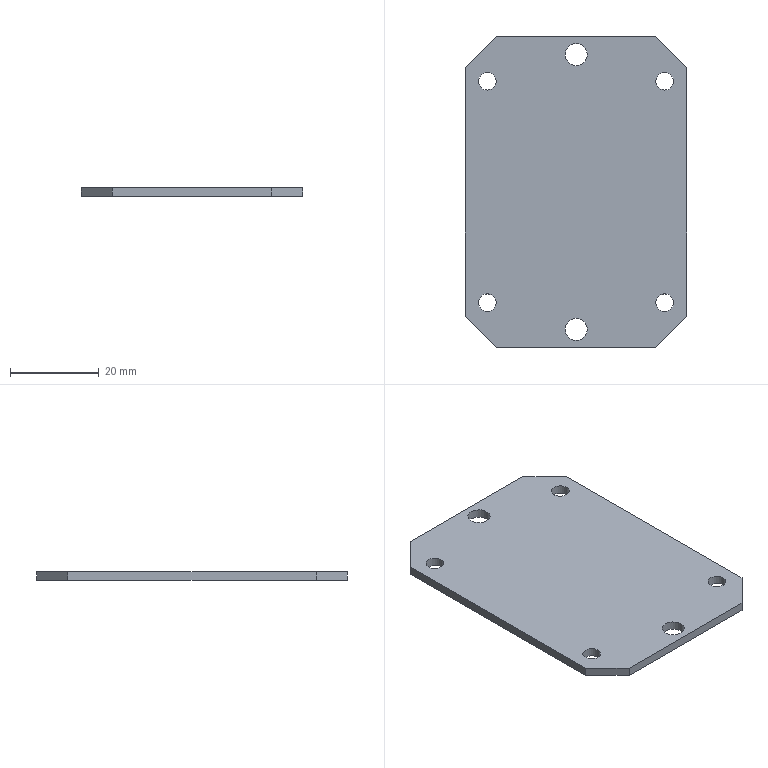Component | NX | PLATE | 1 solid | 16 faces | volume 6625 mm3 | plane 10 | cylinder 6 | commonest cylinder face diameters 4 x4 5 x2